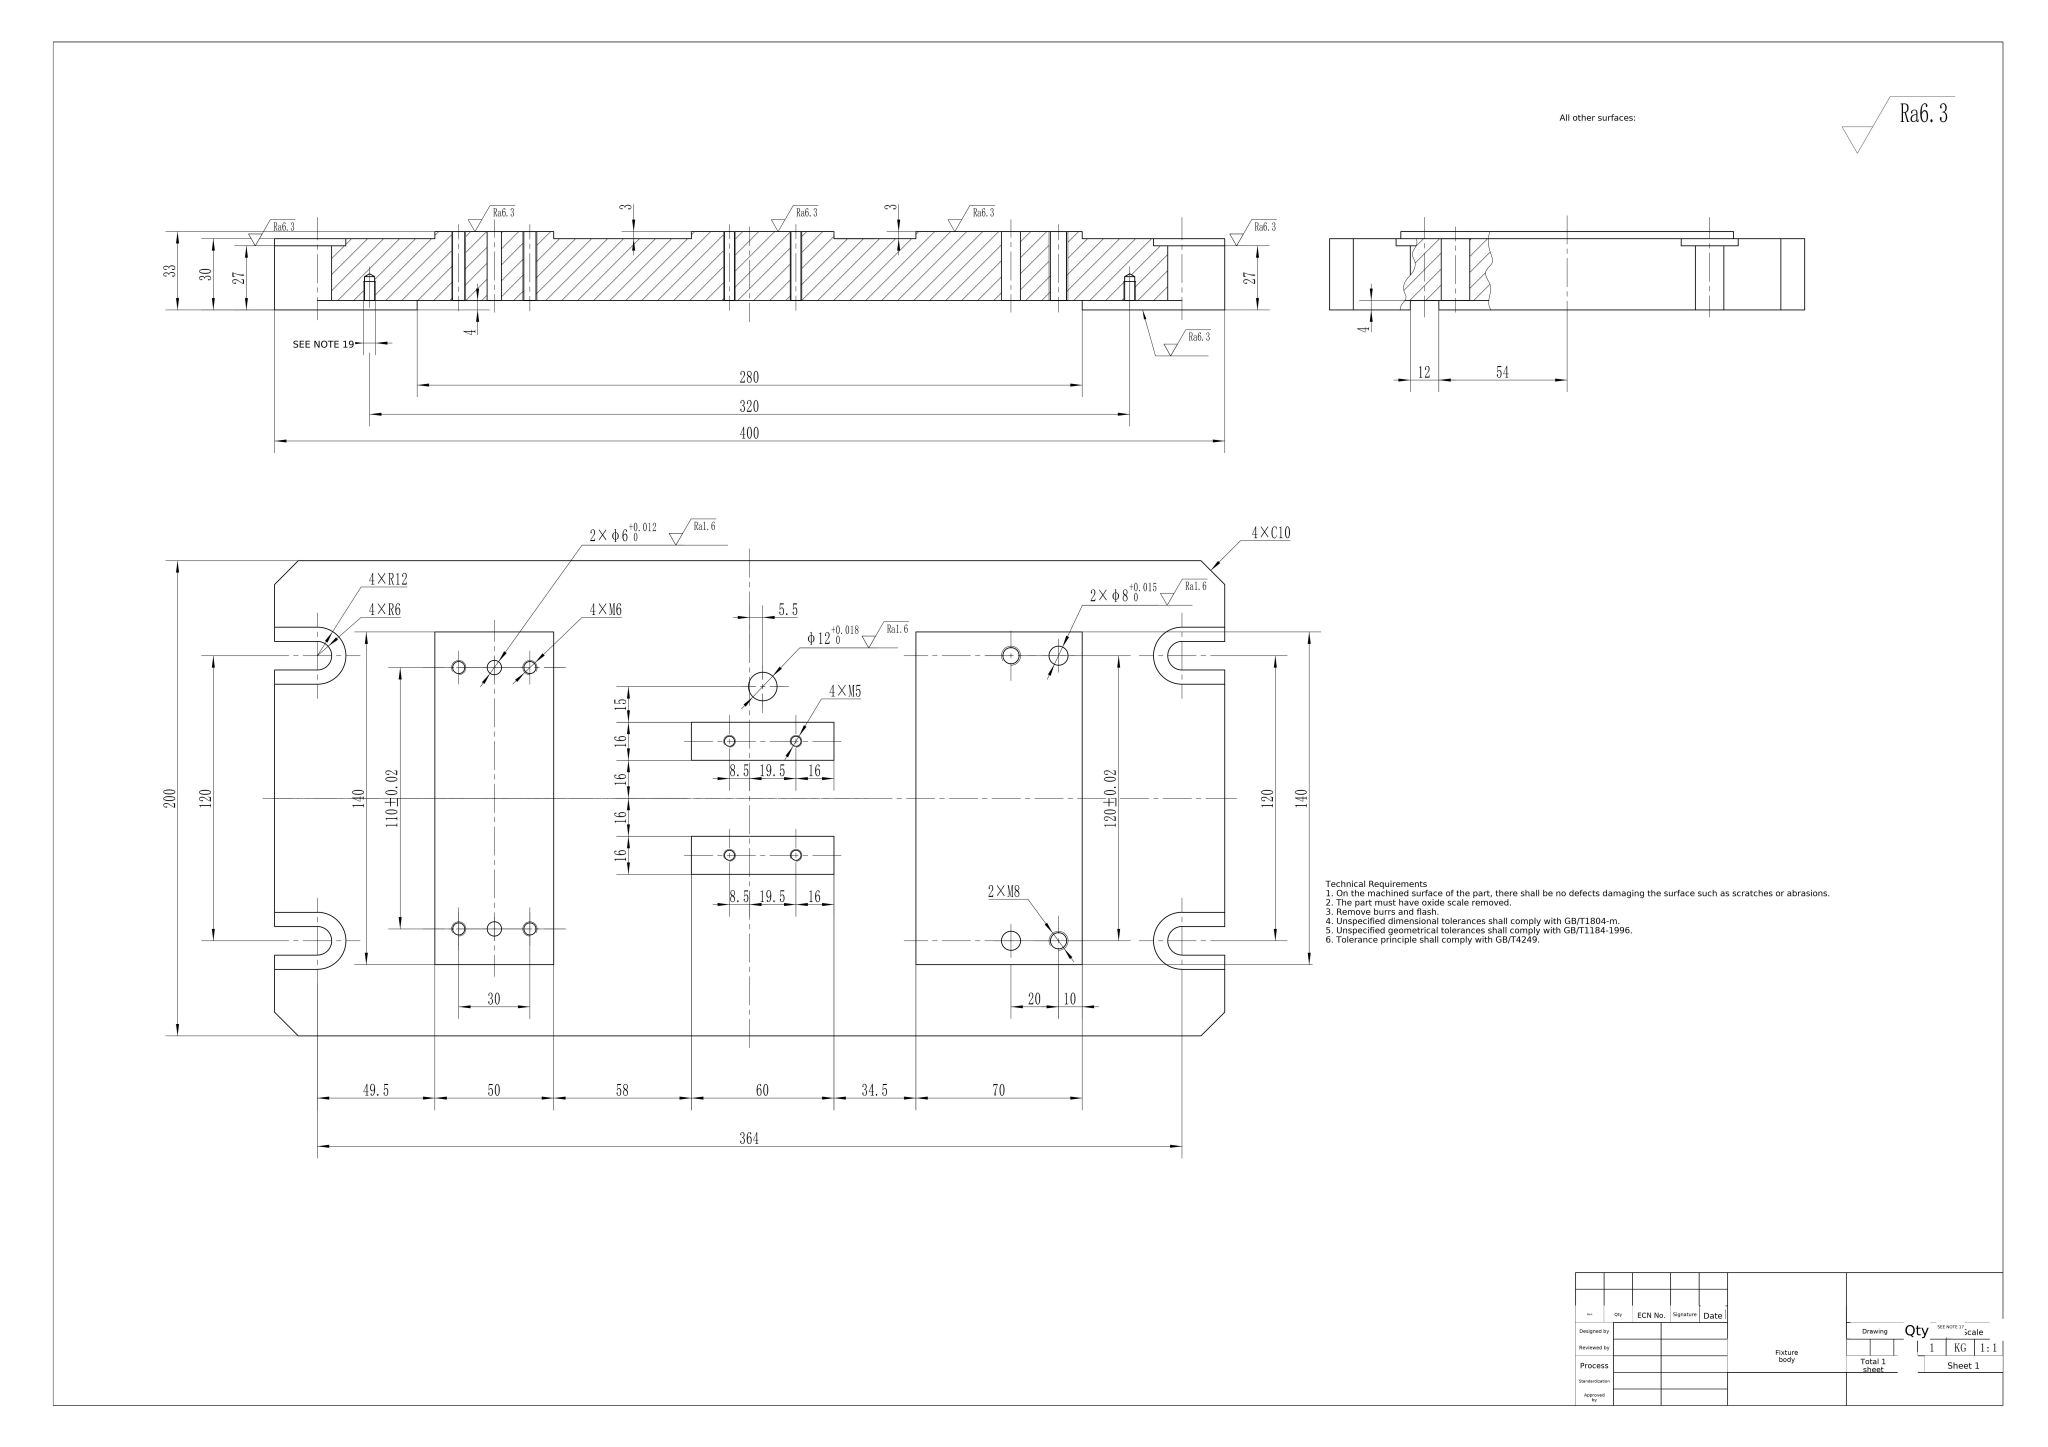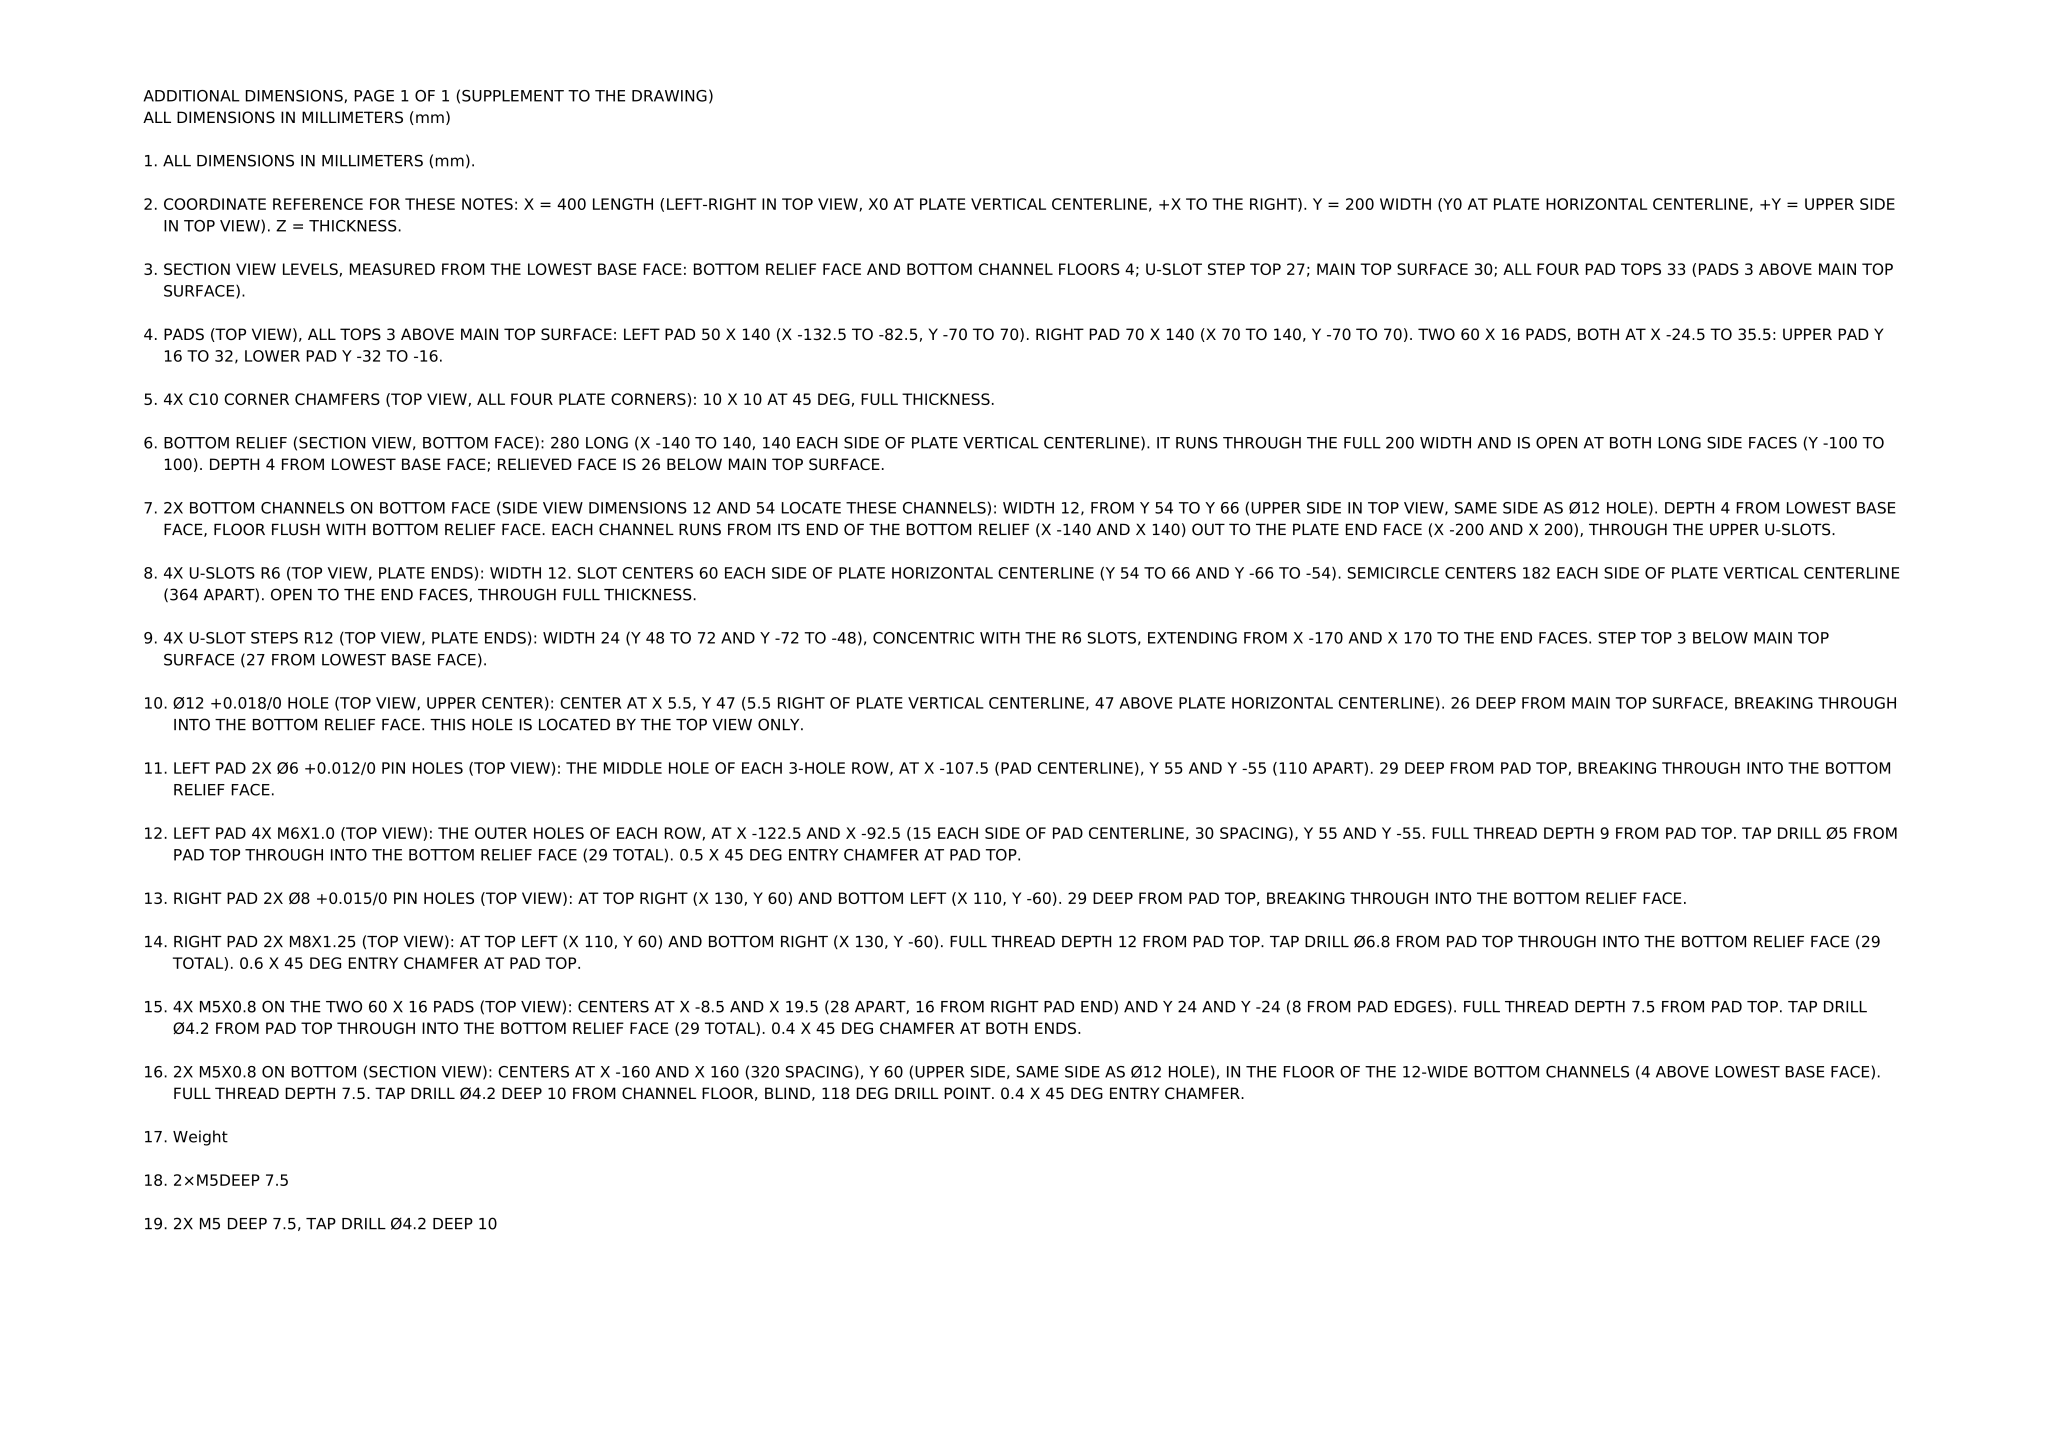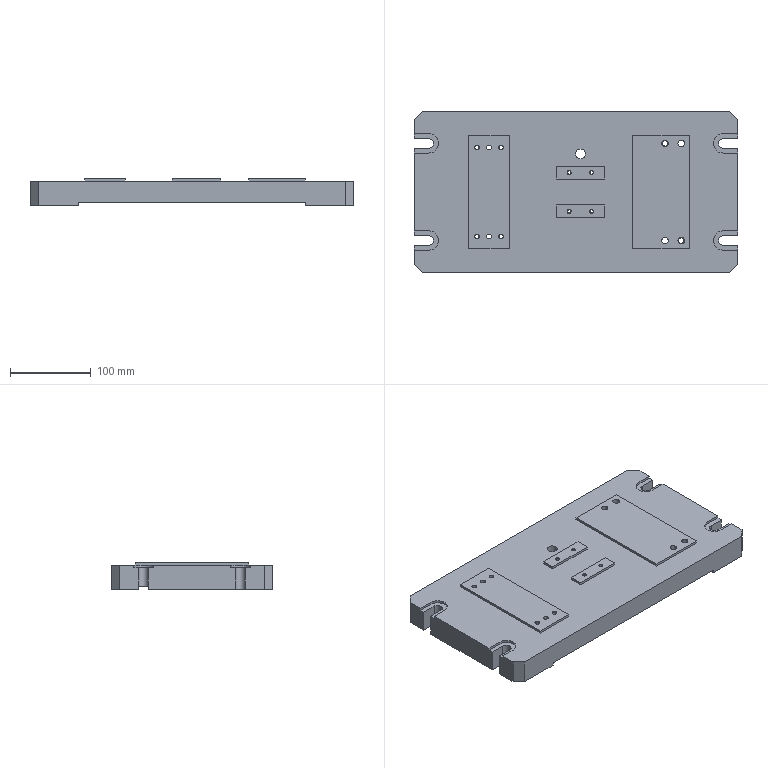Part | NX | mm | 1 solid | 105 faces | box 400 x 200 x 33 mm | volume 2171443 mm3 | plane 62 | cylinder 25 | cone 18 | commonest cylinder face diameters 4.2 x6 12 x5 24 x4 5 x4 6.8 x2 6 x2 8 x2